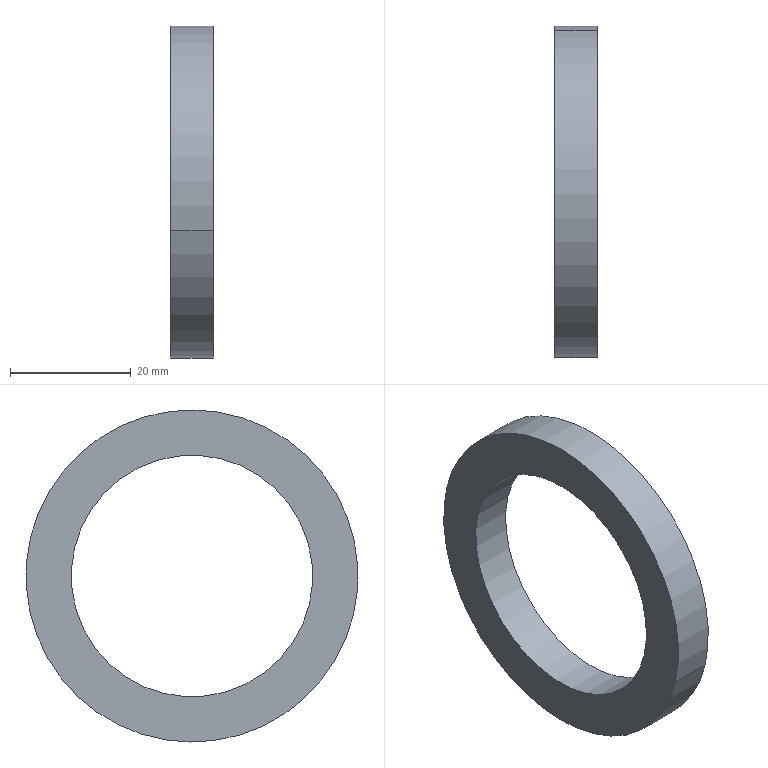Component | SolidWorks | 2-10-10WorkpieceAxisAssembly-1_2-10-7OilSealTC-40X52X7-1 | 1 solid | 12 faces | box 7 x 55 x 55 mm | volume 5745 mm3 | cylinder 8 | plane 4 | commonest cylinder face diameters 44 x2 51 x2 40 x2 55 x2 | material Rubber
build123d program:
from build123d import *

# Parameters (mm, degrees)
SKETCH1_R          = 27.5
SKETCH1_R_2        = 20
EXTRUDE1_DEPTH     = 7
SKETCH2_R          = 25.5
SKETCH2_R_2        = 22
CUT_EXTRUDE1_DEPTH = 4


with BuildPart() as part:
    # Sketch1 → Extrude1 (new body)
    with BuildSketch(Plane(origin=(0, 0, 0), x_dir=(1, 0, 0), z_dir=(0, 1, 0))):
        with Locations(Location((0, 0, 0), (0, 0, 270))):
            Circle(SKETCH1_R)
        with Locations(Location((0, 0, 0), (0, 0, 270))):
            Circle(SKETCH1_R_2, mode=Mode.SUBTRACT)
    extrude(amount=EXTRUDE1_DEPTH)

    # Sketch2 → Cut-Extrude1 (cut)
    with BuildSketch(Plane(origin=(0, 7, 0), x_dir=(1, 0, 0), z_dir=(0, 1, 0))):
        with Locations(Location((0, 0, 0), (0, 0, 270))):
            Circle(SKETCH2_R)
        with Locations(Location((0, 0, 0), (0, 0, 270))):
            Circle(SKETCH2_R_2, mode=Mode.SUBTRACT)
    extrude(amount=-CUT_EXTRUDE1_DEPTH, mode=Mode.SUBTRACT)


solid = part.part

# Placed as in the assembly
solid = solid.moved(Location((-483.809, -4.181, 0), (0, 0, -90)))
STEP:
#1=COLOUR_RGB('',0.7922,0.8196,0.9333);
#2=FILL_AREA_STYLE_COLOUR('',#1);
#3=FILL_AREA_STYLE('',(#2));
#4=SURFACE_STYLE_FILL_AREA(#3);
#5=SURFACE_SIDE_STYLE('',(#4));
#6=SURFACE_STYLE_USAGE(.BOTH.,#5);
#7=PRESENTATION_STYLE_ASSIGNMENT((#6));
#8=CARTESIAN_POINT('',(-18.929,0.6775,0.2024));
#9=VERTEX_POINT('',#8);
#10=CARTESIAN_POINT('',(-18.929,-1.007,-0.2024));
#11=VERTEX_POINT('',#10);
#12=CARTESIAN_POINT('',(-18.929,-0.1646,-0.));
#13=DIRECTION('',(1.,-0.,0.));
#14=DIRECTION('',(0.,0.9723,0.2337));
#15=AXIS2_PLACEMENT_3D('',#12,#13,#14);
#16=CIRCLE('',#15,0.8661);
#17=EDGE_CURVE('',#9,#11,#16,.T.);
#18=ORIENTED_EDGE('',*,*,#17,.T.);
#19=CARTESIAN_POINT('',(-18.772,-1.007,-0.2024));
#20=VERTEX_POINT('',#19);
#21=CARTESIAN_POINT('',(-18.929,-1.007,-0.2024));
#22=DIRECTION('',(1.,-0.,0.));
#23=VECTOR('',#22,39.37);
#24=LINE('',#21,#23);
#25=EDGE_CURVE('',#11,#20,#24,.T.);
#26=ORIENTED_EDGE('',*,*,#25,.T.);
#27=CARTESIAN_POINT('',(-18.772,0.6775,0.2024));
#28=VERTEX_POINT('',#27);
#29=CARTESIAN_POINT('',(-18.772,-0.1646,-0.));
#30=DIRECTION('',(1.,-0.,0.));
#31=DIRECTION('',(0.,0.9723,0.2337));
#32=AXIS2_PLACEMENT_3D('',#29,#30,#31);
#33=CIRCLE('',#32,0.8661);
#34=EDGE_CURVE('',#28,#20,#33,.T.);
#35=ORIENTED_EDGE('',*,*,#34,.F.);
#36=CARTESIAN_POINT('',(-18.929,0.6775,0.2024));
#37=DIRECTION('',(1.,-0.,0.));
#38=VECTOR('',#37,39.37);
#39=LINE('',#36,#38);
#40=EDGE_CURVE('',#9,#28,#39,.T.);
#41=ORIENTED_EDGE('',*,*,#40,.F.);
#42=EDGE_LOOP('',(#18,#26,#35,#41));
#43=FACE_OUTER_BOUND('',#42,.T.);
#44=CARTESIAN_POINT('',(-18.929,-0.1646,-0.));
#45=DIRECTION('',(1.,-0.,0.));
#46=DIRECTION('',(0.,0.9723,0.2337));
#47=AXIS2_PLACEMENT_3D('',#44,#45,#46);
#48=CYLINDRICAL_SURFACE('',#47,0.8661);
#49=ADVANCED_FACE('',(#43),#48,.T.);
#50=CARTESIAN_POINT('',(-18.929,-1.141,-0.2346));
#51=VERTEX_POINT('',#50);
#52=CARTESIAN_POINT('',(-18.929,0.8115,0.2346));
#53=VERTEX_POINT('',#52);
#54=CARTESIAN_POINT('',(-18.929,-0.1646,-0.));
#55=DIRECTION('',(1.,-0.,0.));
#56=DIRECTION('',(0.,0.9723,0.2337));
#57=AXIS2_PLACEMENT_3D('',#54,#55,#56);
#58=CIRCLE('',#57,1.004);
#59=EDGE_CURVE('',#51,#53,#58,.T.);
#60=ORIENTED_EDGE('',*,*,#59,.F.);
#61=CARTESIAN_POINT('',(-18.772,-1.141,-0.2346));
#62=VERTEX_POINT('',#61);
#63=CARTESIAN_POINT('',(-18.929,-1.141,-0.2346));
#64=DIRECTION('',(1.,-0.,0.));
#65=VECTOR('',#64,39.37);
#66=LINE('',#63,#65);
#67=EDGE_CURVE('',#51,#62,#66,.T.);
#68=ORIENTED_EDGE('',*,*,#67,.T.);
#69=CARTESIAN_POINT('',(-18.772,0.8115,0.2346));
#70=VERTEX_POINT('',#69);
#71=CARTESIAN_POINT('',(-18.772,-0.1646,-0.));
#72=DIRECTION('',(1.,-0.,0.));
#73=DIRECTION('',(0.,0.9723,0.2337));
#74=AXIS2_PLACEMENT_3D('',#71,#72,#73);
#75=CIRCLE('',#74,1.004);
#76=EDGE_CURVE('',#62,#70,#75,.T.);
#77=ORIENTED_EDGE('',*,*,#76,.T.);
#78=CARTESIAN_POINT('',(-18.929,0.8115,0.2346));
#79=DIRECTION('',(1.,-0.,0.));
#80=VECTOR('',#79,39.37);
#81=LINE('',#78,#80);
#82=EDGE_CURVE('',#53,#70,#81,.T.);
#83=ORIENTED_EDGE('',*,*,#82,.F.);
#84=EDGE_LOOP('',(#60,#68,#77,#83));
#85=FACE_OUTER_BOUND('',#84,.T.);
#86=CARTESIAN_POINT('',(-18.929,-0.1646,-0.));
#87=DIRECTION('',(1.,-0.,0.));
#88=DIRECTION('',(0.,0.9723,0.2337));
#89=AXIS2_PLACEMENT_3D('',#86,#87,#88);
#90=CYLINDRICAL_SURFACE('',#89,1.004);
#91=ADVANCED_FACE('',(#85),#90,.F.);
#92=CARTESIAN_POINT('',(-18.772,-0.9302,-0.184));
#93=VERTEX_POINT('',#92);
#94=CARTESIAN_POINT('',(-18.772,0.601,0.184));
#95=VERTEX_POINT('',#94);
#96=CARTESIAN_POINT('',(-18.772,-0.1646,-0.));
#97=DIRECTION('',(1.,-0.,0.));
#98=DIRECTION('',(0.,0.9723,0.2337));
#99=AXIS2_PLACEMENT_3D('',#96,#97,#98);
#100=CIRCLE('',#99,0.7874);
#101=EDGE_CURVE('',#93,#95,#100,.T.);
#102=ORIENTED_EDGE('',*,*,#101,.T.);
#103=CARTESIAN_POINT('',(-19.048,0.601,0.184));
#104=VERTEX_POINT('',#103);
#105=CARTESIAN_POINT('',(-18.772,0.601,0.184));
#106=DIRECTION('',(-1.,0.,-0.));
#107=VECTOR('',#106,39.37);
#108=LINE('',#105,#107);
#109=EDGE_CURVE('',#95,#104,#108,.T.);
#110=ORIENTED_EDGE('',*,*,#109,.T.);
#111=CARTESIAN_POINT('',(-19.048,-0.9302,-0.184));
#112=VERTEX_POINT('',#111);
#113=CARTESIAN_POINT('',(-19.048,-0.1646,-0.));
#114=DIRECTION('',(1.,-0.,0.));
#115=DIRECTION('',(0.,0.9723,0.2337));
#116=AXIS2_PLACEMENT_3D('',#113,#114,#115);
#117=CIRCLE('',#116,0.7874);
#118=EDGE_CURVE('',#112,#104,#117,.T.);
#119=ORIENTED_EDGE('',*,*,#118,.F.);
#120=CARTESIAN_POINT('',(-18.772,-0.9302,-0.184));
#121=DIRECTION('',(-1.,0.,-0.));
#122=VECTOR('',#121,39.37);
#123=LINE('',#120,#122);
#124=EDGE_CURVE('',#93,#112,#123,.T.);
#125=ORIENTED_EDGE('',*,*,#124,.F.);
#126=EDGE_LOOP('',(#102,#110,#119,#125));
#127=FACE_OUTER_BOUND('',#126,.T.);
#128=CARTESIAN_POINT('',(-18.772,-0.1646,-0.));
#129=DIRECTION('',(-1.,0.,-0.));
#130=DIRECTION('',(0.,-0.9723,-0.2337));
#131=AXIS2_PLACEMENT_3D('',#128,#129,#130);
#132=CYLINDRICAL_SURFACE('',#131,0.7874);
#133=ADVANCED_FACE('',(#127),#132,.F.);
#134=CARTESIAN_POINT('',(-18.772,0.8881,0.253));
#135=VERTEX_POINT('',#134);
#136=CARTESIAN_POINT('',(-18.772,-1.217,-0.253));
#137=VERTEX_POINT('',#136);
#138=CARTESIAN_POINT('',(-18.772,-0.1646,-0.));
#139=DIRECTION('',(1.,-0.,0.));
#140=DIRECTION('',(0.,0.9723,0.2337));
#141=AXIS2_PLACEMENT_3D('',#138,#139,#140);
#142=CIRCLE('',#141,1.083);
#143=EDGE_CURVE('',#135,#137,#142,.T.);
#144=ORIENTED_EDGE('',*,*,#143,.F.);
#145=CARTESIAN_POINT('',(-19.048,0.8881,0.253));
#146=VERTEX_POINT('',#145);
#147=CARTESIAN_POINT('',(-18.772,0.8881,0.253));
#148=DIRECTION('',(-1.,0.,-0.));
#149=VECTOR('',#148,39.37);
#150=LINE('',#147,#149);
#151=EDGE_CURVE('',#135,#146,#150,.T.);
#152=ORIENTED_EDGE('',*,*,#151,.T.);
#153=CARTESIAN_POINT('',(-19.048,-1.217,-0.253));
#154=VERTEX_POINT('',#153);
#155=CARTESIAN_POINT('',(-19.048,-0.1646,-0.));
#156=DIRECTION('',(1.,-0.,0.));
#157=DIRECTION('',(0.,0.9723,0.2337));
#158=AXIS2_PLACEMENT_3D('',#155,#156,#157);
#159=CIRCLE('',#158,1.083);
#160=EDGE_CURVE('',#146,#154,#159,.T.);
#161=ORIENTED_EDGE('',*,*,#160,.T.);
#162=CARTESIAN_POINT('',(-18.772,-1.217,-0.253));
#163=DIRECTION('',(-1.,0.,-0.));
#164=VECTOR('',#163,39.37);
#165=LINE('',#162,#164);
#166=EDGE_CURVE('',#137,#154,#165,.T.);
#167=ORIENTED_EDGE('',*,*,#166,.F.);
#168=EDGE_LOOP('',(#144,#152,#161,#167));
#169=FACE_OUTER_BOUND('',#168,.T.);
#170=CARTESIAN_POINT('',(-18.772,-0.1646,-0.));
#171=DIRECTION('',(-1.,0.,-0.));
#172=DIRECTION('',(0.,-0.9723,-0.2337));
#173=AXIS2_PLACEMENT_3D('',#170,#171,#172);
#174=CYLINDRICAL_SURFACE('',#173,1.083);
#175=ADVANCED_FACE('',(#169),#174,.T.);
#176=ORIENTED_EDGE('',*,*,#101,.F.);
#177=CARTESIAN_POINT('',(-18.772,-0.1646,-0.));
#178=DIRECTION('',(1.,-0.,0.));
#179=DIRECTION('',(0.,0.9723,0.2337));
#180=AXIS2_PLACEMENT_3D('',#177,#178,#179);
#181=CIRCLE('',#180,0.7874);
#182=EDGE_CURVE('',#95,#93,#181,.T.);
#183=ORIENTED_EDGE('',*,*,#182,.F.);
#184=EDGE_LOOP('',(#176,#183));
#185=FACE_BOUND('',#184,.T.);
#186=ORIENTED_EDGE('',*,*,#34,.T.);
#187=CARTESIAN_POINT('',(-18.772,-0.1646,-0.));
#188=DIRECTION('',(1.,-0.,0.));
#189=DIRECTION('',(0.,0.9723,0.2337));
#190=AXIS2_PLACEMENT_3D('',#187,#188,#189);
#191=CIRCLE('',#190,0.8661);
#192=EDGE_CURVE('',#20,#28,#191,.T.);
#193=ORIENTED_EDGE('',*,*,#192,.T.);
#194=EDGE_LOOP('',(#186,#193));
#195=FACE_OUTER_BOUND('',#194,.T.);
#196=CARTESIAN_POINT('',(-18.772,-0.1646,-0.));
#197=DIRECTION('',(1.,-0.,0.));
#198=DIRECTION('',(0.,0.9723,0.2337));
#199=AXIS2_PLACEMENT_3D('',#196,#197,#198);
#200=PLANE('',#199);
#201=ADVANCED_FACE('',(#185,#195),#200,.T.);
#202=CARTESIAN_POINT('',(-18.772,-0.1646,-0.));
#203=DIRECTION('',(1.,-0.,0.));
#204=DIRECTION('',(0.,0.9723,0.2337));
#205=AXIS2_PLACEMENT_3D('',#202,#203,#204);
#206=CIRCLE('',#205,1.004);
#207=EDGE_CURVE('',#70,#62,#206,.T.);
#208=ORIENTED_EDGE('',*,*,#207,.F.);
#209=ORIENTED_EDGE('',*,*,#76,.F.);
#210=EDGE_LOOP('',(#208,#209));
#211=FACE_BOUND('',#210,.T.);
#212=CARTESIAN_POINT('',(-18.772,-0.1646,-0.));
#213=DIRECTION('',(1.,-0.,0.));
#214=DIRECTION('',(0.,0.9723,0.2337));
#215=AXIS2_PLACEMENT_3D('',#212,#213,#214);
#216=CIRCLE('',#215,1.083);
#217=EDGE_CURVE('',#137,#135,#216,.T.);
#218=ORIENTED_EDGE('',*,*,#217,.T.);
#219=ORIENTED_EDGE('',*,*,#143,.T.);
#220=EDGE_LOOP('',(#218,#219));
#221=FACE_OUTER_BOUND('',#220,.T.);
#222=CARTESIAN_POINT('',(-18.772,-0.1646,-0.));
#223=DIRECTION('',(1.,-0.,0.));
#224=DIRECTION('',(0.,0.9723,0.2337));
#225=AXIS2_PLACEMENT_3D('',#222,#223,#224);
#226=PLANE('',#225);
#227=ADVANCED_FACE('',(#211,#221),#226,.T.);
#228=CARTESIAN_POINT('',(-19.048,-0.1646,-0.));
#229=DIRECTION('',(1.,-0.,0.));
#230=DIRECTION('',(0.,0.9723,0.2337));
#231=AXIS2_PLACEMENT_3D('',#228,#229,#230);
#232=CIRCLE('',#231,1.083);
#233=EDGE_CURVE('',#154,#146,#232,.T.);
#234=ORIENTED_EDGE('',*,*,#233,.F.);
#235=ORIENTED_EDGE('',*,*,#160,.F.);
#236=EDGE_LOOP('',(#234,#235));
#237=FACE_OUTER_BOUND('',#236,.T.);
#238=ORIENTED_EDGE('',*,*,#118,.T.);
#239=CARTESIAN_POINT('',(-19.048,-0.1646,-0.));
#240=DIRECTION('',(1.,-0.,0.));
#241=DIRECTION('',(0.,0.9723,0.2337));
#242=AXIS2_PLACEMENT_3D('',#239,#240,#241);
#243=CIRCLE('',#242,0.7874);
#244=EDGE_CURVE('',#104,#112,#243,.T.);
#245=ORIENTED_EDGE('',*,*,#244,.T.);
#246=EDGE_LOOP('',(#238,#245));
#247=FACE_BOUND('',#246,.T.);
#248=CARTESIAN_POINT('',(-19.048,-0.1646,-0.));
#249=DIRECTION('',(1.,-0.,0.));
#250=DIRECTION('',(0.,0.9723,0.2337));
#251=AXIS2_PLACEMENT_3D('',#248,#249,#250);
#252=PLANE('',#251);
#253=ADVANCED_FACE('',(#237,#247),#252,.F.);
#254=ORIENTED_EDGE('',*,*,#151,.F.);
#255=ORIENTED_EDGE('',*,*,#217,.F.);
#256=ORIENTED_EDGE('',*,*,#166,.T.);
#257=ORIENTED_EDGE('',*,*,#233,.T.);
#258=EDGE_LOOP('',(#254,#255,#256,#257));
#259=FACE_OUTER_BOUND('',#258,.T.);
#260=CARTESIAN_POINT('',(-18.772,-0.1646,-0.));
#261=DIRECTION('',(-1.,0.,-0.));
#262=DIRECTION('',(0.,-0.9723,-0.2337));
#263=AXIS2_PLACEMENT_3D('',#260,#261,#262);
#264=CYLINDRICAL_SURFACE('',#263,1.083);
#265=ADVANCED_FACE('',(#259),#264,.T.);
#266=ORIENTED_EDGE('',*,*,#109,.F.);
#267=ORIENTED_EDGE('',*,*,#182,.T.);
#268=ORIENTED_EDGE('',*,*,#124,.T.);
#269=ORIENTED_EDGE('',*,*,#244,.F.);
#270=EDGE_LOOP('',(#266,#267,#268,#269));
#271=FACE_OUTER_BOUND('',#270,.T.);
#272=CARTESIAN_POINT('',(-18.772,-0.1646,-0.));
#273=DIRECTION('',(-1.,0.,-0.));
#274=DIRECTION('',(0.,-0.9723,-0.2337));
#275=AXIS2_PLACEMENT_3D('',#272,#273,#274);
#276=CYLINDRICAL_SURFACE('',#275,0.7874);
#277=ADVANCED_FACE('',(#271),#276,.F.);
#278=ORIENTED_EDGE('',*,*,#67,.F.);
#279=CARTESIAN_POINT('',(-18.929,-0.1646,-0.));
#280=DIRECTION('',(1.,-0.,0.));
#281=DIRECTION('',(0.,0.9723,0.2337));
#282=AXIS2_PLACEMENT_3D('',#279,#280,#281);
#283=CIRCLE('',#282,1.004);
#284=EDGE_CURVE('',#53,#51,#283,.T.);
#285=ORIENTED_EDGE('',*,*,#284,.F.);
#286=ORIENTED_EDGE('',*,*,#82,.T.);
#287=ORIENTED_EDGE('',*,*,#207,.T.);
#288=EDGE_LOOP('',(#278,#285,#286,#287));
#289=FACE_OUTER_BOUND('',#288,.T.);
#290=CARTESIAN_POINT('',(-18.929,-0.1646,-0.));
#291=DIRECTION('',(1.,-0.,0.));
#292=DIRECTION('',(0.,0.9723,0.2337));
#293=AXIS2_PLACEMENT_3D('',#290,#291,#292);
#294=CYLINDRICAL_SURFACE('',#293,1.004);
#295=ADVANCED_FACE('',(#289),#294,.F.);
#296=ORIENTED_EDGE('',*,*,#17,.F.);
#297=CARTESIAN_POINT('',(-18.929,-0.1646,-0.));
#298=DIRECTION('',(1.,-0.,0.));
#299=DIRECTION('',(0.,0.9723,0.2337));
#300=AXIS2_PLACEMENT_3D('',#297,#298,#299);
#301=CIRCLE('',#300,0.8661);
#302=EDGE_CURVE('',#11,#9,#301,.T.);
#303=ORIENTED_EDGE('',*,*,#302,.F.);
#304=EDGE_LOOP('',(#296,#303));
#305=FACE_BOUND('',#304,.T.);
#306=ORIENTED_EDGE('',*,*,#284,.T.);
#307=ORIENTED_EDGE('',*,*,#59,.T.);
#308=EDGE_LOOP('',(#306,#307));
#309=FACE_OUTER_BOUND('',#308,.T.);
#310=CARTESIAN_POINT('',(-18.929,-0.1646,-0.));
#311=DIRECTION('',(1.,-0.,0.));
#312=DIRECTION('',(0.,0.9723,0.2337));
#313=AXIS2_PLACEMENT_3D('',#310,#311,#312);
#314=PLANE('',#313);
#315=ADVANCED_FACE('',(#305,#309),#314,.T.);
#316=ORIENTED_EDGE('',*,*,#25,.F.);
#317=ORIENTED_EDGE('',*,*,#302,.T.);
#318=ORIENTED_EDGE('',*,*,#40,.T.);
#319=ORIENTED_EDGE('',*,*,#192,.F.);
#320=EDGE_LOOP('',(#316,#317,#318,#319));
#321=FACE_OUTER_BOUND('',#320,.T.);
#322=CARTESIAN_POINT('',(-18.929,-0.1646,-0.));
#323=DIRECTION('',(1.,-0.,0.));
#324=DIRECTION('',(0.,0.9723,0.2337));
#325=AXIS2_PLACEMENT_3D('',#322,#323,#324);
#326=CYLINDRICAL_SURFACE('',#325,0.8661);
#327=ADVANCED_FACE('',(#321),#326,.T.);
#328=CLOSED_SHELL('',(#49,#91,#133,#175,#201,#227,#253,#265,#277,#295,#315,#327));
#329=MANIFOLD_SOLID_BREP('',#328);
#330=STYLED_ITEM('',(#7),#329);
#331=PRESENTATION_LAYER_ASSIGNMENT('','',(#330));
#332=(LENGTH_UNIT()NAMED_UNIT(*)SI_UNIT($,.METRE.));
#333=LENGTH_MEASURE_WITH_UNIT(LENGTH_MEASURE(0.0254),#332);
#334=DIMENSIONAL_EXPONENTS(1.,0.,0.,0.,0.,0.,0.);
#335=(CONVERSION_BASED_UNIT('',#333)LENGTH_UNIT()NAMED_UNIT(#334));
#336=UNCERTAINTY_MEASURE_WITH_UNIT(LENGTH_MEASURE(0.00001),#335,'','');
#337=(NAMED_UNIT(*)PLANE_ANGLE_UNIT()SI_UNIT($,.RADIAN.));
#338=(NAMED_UNIT(*)SI_UNIT($,.STERADIAN.)SOLID_ANGLE_UNIT());
#339=(GEOMETRIC_REPRESENTATION_CONTEXT(3)GLOBAL_UNCERTAINTY_ASSIGNED_CONTEXT((#336))GLOBAL_UNIT_ASSIGNED_CONTEXT((#335,#337,#338))REPRESENTATION_CONTEXT('',''));
#340=MECHANICAL_DESIGN_GEOMETRIC_PRESENTATION_REPRESENTATION('',(#330),#339);
#341=CARTESIAN_POINT('',(0.,0.,0.));
#342=DIRECTION('',(0.,0.,1.));
#343=DIRECTION('',(1.,0.,0.));
#344=AXIS2_PLACEMENT_3D('',#341,#342,#343);
#345=(LENGTH_UNIT()NAMED_UNIT(*)SI_UNIT($,.METRE.));
#346=LENGTH_MEASURE_WITH_UNIT(LENGTH_MEASURE(0.0254),#345);
#347=DIMENSIONAL_EXPONENTS(1.,0.,0.,0.,0.,0.,0.);
#348=(CONVERSION_BASED_UNIT('',#346)LENGTH_UNIT()NAMED_UNIT(#347));
#349=UNCERTAINTY_MEASURE_WITH_UNIT(LENGTH_MEASURE(0.00001),#348,'','');
#350=(NAMED_UNIT(*)PLANE_ANGLE_UNIT()SI_UNIT($,.RADIAN.));
#351=(NAMED_UNIT(*)SI_UNIT($,.STERADIAN.)SOLID_ANGLE_UNIT());
#352=(GEOMETRIC_REPRESENTATION_CONTEXT(3)GLOBAL_UNCERTAINTY_ASSIGNED_CONTEXT((#349))GLOBAL_UNIT_ASSIGNED_CONTEXT((#348,#350,#351))REPRESENTATION_CONTEXT('',''));
#353=ADVANCED_BREP_SHAPE_REPRESENTATION('',(#329,#344),#352);